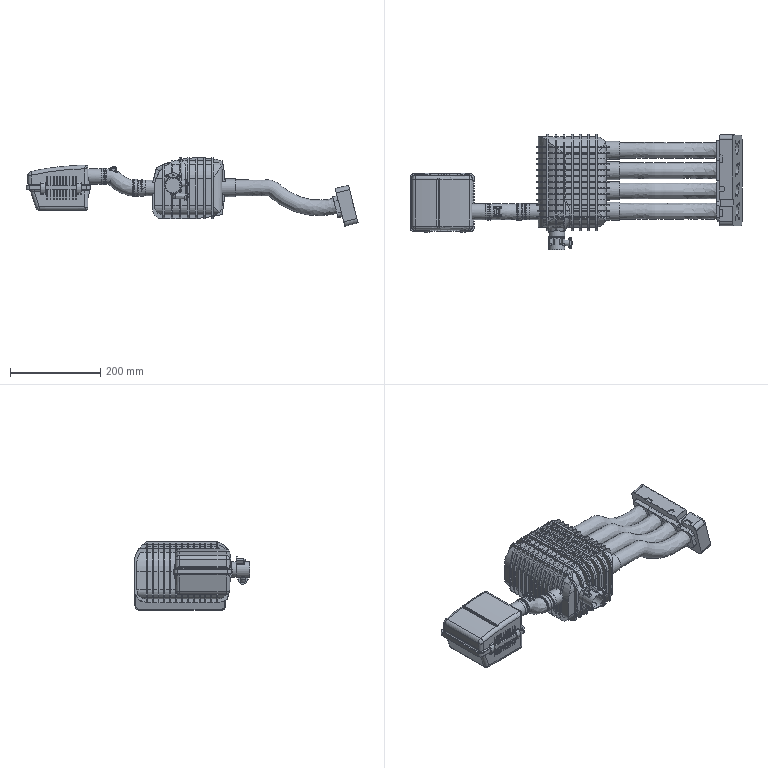Assembly | NX | mm | 5 component files | 8 solids | 1919 faces | box 736.35 x 255.56 x 152.03 mm | volume 5408139 mm3 | plane 1271 | cylinder 542 | spline 66 | torus 30 | sphere 10 | commonest cylinder face diameters 410.429 x101 40 x64 594.21 x51 120 x48 80 x38 4 x25 2 x25 16 x24
Bill of materials:
unnamed part 1 | 1 |  | Rounded rectangular box-like hollow body covered with many parallel thin external ribs/fins and a top lattice of crossing ribs; four parallel open-ended round tubular stubs protrude in a row from one long side, with a single larger tubular stub on each short end and one more stub on a bottom/side face.
unnamed part 2 | 1 |  | Four parallel, identically shaped S-curved round tubes terminating in a single thick rectangular flat flange plate with rounded corners; the flange has one circular through-opening per tube plus small holes arranged around them, and a notch/step on one long edge.
unnamed part 3 | 1 |  | Single round hollow tube with an offset S-shaped bend between two straight sections, with several raised circumferential bands/beads near each end and a small rectangular raised boss with stepped tab and small holes on the outer surface near one end.
unnamed part 4 | 1 |  | Short large-diameter open cylindrical sleeve with a winged/pentagonal-shaped raised pocket on one side, connected by two smaller cylindrical side arms (one straight, one elbowed) to an elongated rounded-end plate carrying two circular stepped bosses.
unnamed part 5 | 1 |  | Rounded rectangular enclosure-like body with a slightly sloped/domed top divided by a shallow longitudinal groove, a peripheral flange/lip around the mid-height, rows of vertical slot-like recesses on the sides above and below the lip, clip-like tabs on two sides, and one large circular opening on one side wall.
Mates:
1. concentric | intake_pipe 1 arc | air_filter_housing 1 edge
2. concentric | intake_pipe 1 edge | pressure_chamber 1 edge
3. concentric | e_throttle 1 arc | pressure_chamber 1 edge
4. concentric | pipe_1_4 1 arc | pressure_chamber 1 edge